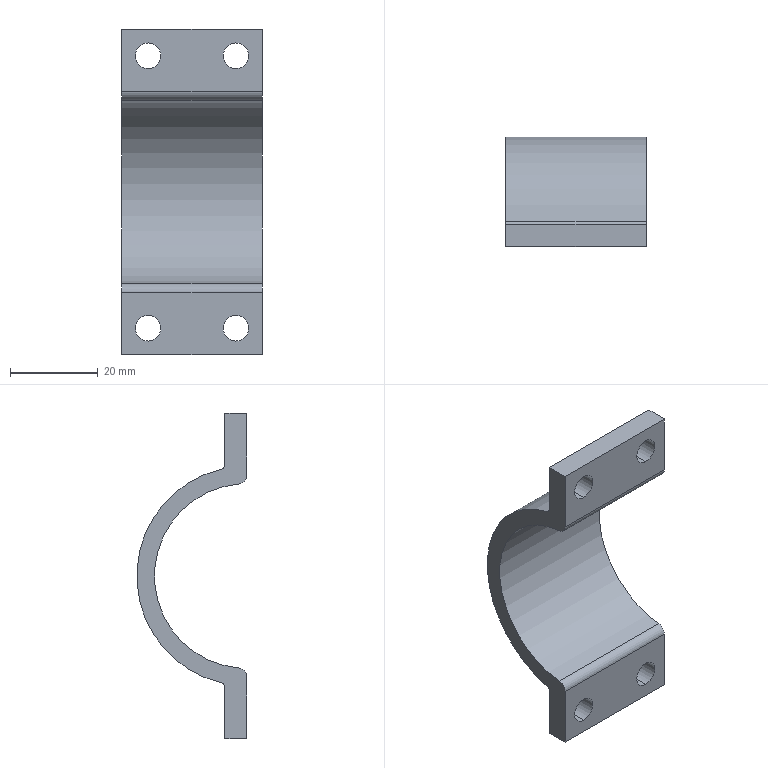Component | SolidWorks | Cover-1 | 1 solid | 22 faces | box 32 x 25 x 74 mm | volume 12574 mm3 | cylinder 14 | plane 8 | commonest cylinder face diameters 5.8 x8 2 x2 4 x2 42 x1 50 x1 | material 6061 Alloy
build123d program:
from build123d import *

# Parameters (mm, degrees)
BOSS_EXTRUDE2_DEPTH = 16
SKETCH2_R           = 2.9
CUT_EXTRUDE1_DEPTH  = 46
FILLET1_R           = 1
FILLET2_R           = 2


with BuildPart() as part:
    # Sketch1 → Boss-Extrude2 (new, symmetric)
    with BuildSketch(Plane(origin=(0, 0, 0), x_dir=(0, 0, -1), z_dir=(1, 0, 0))):
        with BuildLine():
            Line((-21, 0), (-37, 0))
            Line((-37, 0), (-37, 5))
            Line((-37, 5), (-24.495, 5))
            ThreePointArc((-24.495, 5), (0, 25), (24.495, 5))
            Line((24.495, 5), (37, 5))
            Line((37, 5), (37, 0))
            Line((37, 0), (21, 0))
            ThreePointArc((21, 0), (0, 21), (-21, 0))
        make_face()
    extrude(amount=BOSS_EXTRUDE2_DEPTH, both=True)

    # Sketch2 → Cut-Extrude1 (cut, through all)
    with BuildSketch(Plane(origin=(0, 5, 0), x_dir=(1, 0, 0), z_dir=(0, 1, 0))):
        with Locations(Location((-10, -31, 0), (0, 0, 270))):
            Circle(SKETCH2_R)
        with Locations(Location((10, -31, 0), (0, 0, 90))):
            Circle(SKETCH2_R)
    cut_extrude1 = extrude(amount=-CUT_EXTRUDE1_DEPTH, mode=Mode.SUBTRACT)

    # Mirror1: Cut-Extrude1 across plane
    add(cut_extrude1.mirror(Plane.XY), mode=Mode.SUBTRACT)

    # Fillet1
    fillet1_edges = [part.edges().sort_by_distance(p)[0] for p in [
        (0, 5, 24.495),
        (0, 5, -24.495),
    ]]
    fillet(fillet1_edges, radius=FILLET1_R)

    # Fillet2
    fillet2_edges = [part.edges().sort_by_distance(p)[0] for p in [
        (0, 0, -21),
        (0, 0, 21),
    ]]
    fillet(fillet2_edges, radius=FILLET2_R)


solid = part.part

# Placed as in the assembly
solid = solid.moved(Location((-249.428, 167.796, 284.382), (0, 0, 0)))